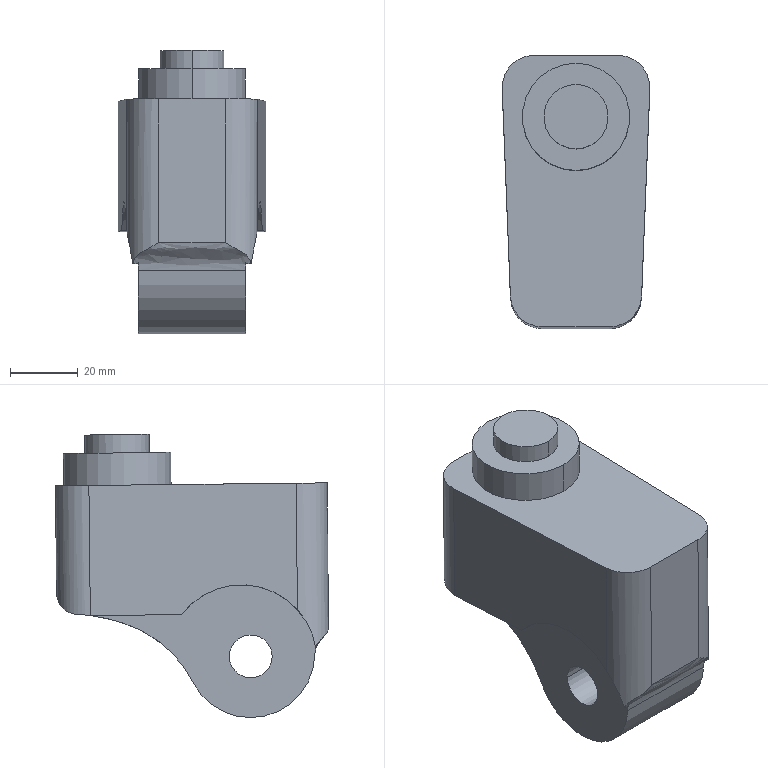Component | NX | CONNECTOR | 1 solid | 27 faces | box 43.68 x 80.82 x 83.81 mm | volume 165748 mm3 | cylinder 14 | plane 11 | spline 2 | commonest cylinder face diameters 19.05 x6 12.7 x3 31.75 x2 44.533 x2 38.1 x1
STEP:
#1=VALUE_REPRESENTATION_ITEM('',COUNT_MEASURE(0.));
#2=(LENGTH_UNIT()NAMED_UNIT(*)SI_UNIT(.MILLI.,.METRE.));
#3=UNCERTAINTY_MEASURE_WITH_UNIT(LENGTH_MEASURE(0.0508),#2,'','');
#4=(NAMED_UNIT(*)PLANE_ANGLE_UNIT()SI_UNIT($,.RADIAN.));
#5=PLANE_ANGLE_MEASURE_WITH_UNIT(PLANE_ANGLE_MEASURE(0.01745),#4);
#6=DIMENSIONAL_EXPONENTS(0.,0.,0.,0.,0.,0.,0.);
#7=(CONVERSION_BASED_UNIT('',#5)NAMED_UNIT(#6)PLANE_ANGLE_UNIT());
#8=(NAMED_UNIT(*)SI_UNIT($,.STERADIAN.)SOLID_ANGLE_UNIT());
#9=(GEOMETRIC_REPRESENTATION_CONTEXT(3)GLOBAL_UNCERTAINTY_ASSIGNED_CONTEXT((#3))GLOBAL_UNIT_ASSIGNED_CONTEXT((#2,#7,#8))REPRESENTATION_CONTEXT('',''));
#10=REPRESENTATION('',(#1),#9);
#11=VALUE_REPRESENTATION_ITEM('',COUNT_MEASURE(0.));
#12=REPRESENTATION('',(#11),#9);
#13=CARTESIAN_POINT('',(0.,0.,0.));
#14=DIRECTION('',(0.,0.,1.));
#15=DIRECTION('',(1.,0.,0.));
#16=AXIS2_PLACEMENT_3D('',#13,#14,#15);
#17=SHAPE_REPRESENTATION('',(#16),#9);
#18=CARTESIAN_POINT('',(-0.,49.153,252.991));
#19=VERTEX_POINT('',#18);
#20=CARTESIAN_POINT('',(-0.,49.095,247.591));
#21=VERTEX_POINT('',#20);
#22=CARTESIAN_POINT('',(-0.,49.371,272.99));
#23=DIRECTION('',(0.,-0.01088,-0.9999));
#24=VECTOR('',#23,1.);
#25=LINE('',#22,#24);
#26=EDGE_CURVE('',#19,#21,#25,.T.);
#27=ORIENTED_EDGE('',*,*,#26,.F.);
#28=CARTESIAN_POINT('',(-0.,30.104,253.198));
#29=VERTEX_POINT('',#28);
#30=CARTESIAN_POINT('',(-0.,39.629,253.095));
#31=DIRECTION('',(0.,-0.01088,-0.9999));
#32=DIRECTION('',(0.,-0.9999,0.01088));
#33=AXIS2_PLACEMENT_3D('',#30,#31,#32);
#34=CIRCLE('',#33,9.525);
#35=EDGE_CURVE('',#19,#29,#34,.T.);
#36=ORIENTED_EDGE('',*,*,#35,.T.);
#37=CARTESIAN_POINT('',(-0.,30.046,247.799));
#38=VERTEX_POINT('',#37);
#39=CARTESIAN_POINT('',(-0.,30.322,273.197));
#40=DIRECTION('',(0.,-0.01088,-0.9999));
#41=VECTOR('',#40,1.);
#42=LINE('',#39,#41);
#43=EDGE_CURVE('',#29,#38,#42,.T.);
#44=ORIENTED_EDGE('',*,*,#43,.T.);
#45=CARTESIAN_POINT('',(-0.,39.57,247.695));
#46=DIRECTION('',(-0.,0.01088,0.9999));
#47=DIRECTION('',(0.,-0.9999,0.01088));
#48=AXIS2_PLACEMENT_3D('',#45,#46,#47);
#49=CIRCLE('',#48,9.525);
#50=EDGE_CURVE('',#38,#21,#49,.T.);
#51=ORIENTED_EDGE('',*,*,#50,.T.);
#52=EDGE_LOOP('',(#27,#36,#44,#51));
#53=FACE_OUTER_BOUND('',#52,.T.);
#54=CARTESIAN_POINT('',(-0.,39.847,273.093));
#55=DIRECTION('',(0.,-0.01088,-0.9999));
#56=DIRECTION('',(0.,-0.9999,0.01088));
#57=AXIS2_PLACEMENT_3D('',#54,#55,#56);
#58=CYLINDRICAL_SURFACE('',#57,9.525);
#59=ADVANCED_FACE('',(#53),#58,.T.);
#60=ORIENTED_EDGE('',*,*,#43,.F.);
#61=CARTESIAN_POINT('',(-0.,39.629,253.095));
#62=DIRECTION('',(0.,-0.01088,-0.9999));
#63=DIRECTION('',(0.,-0.9999,0.01088));
#64=AXIS2_PLACEMENT_3D('',#61,#62,#63);
#65=CIRCLE('',#64,9.525);
#66=EDGE_CURVE('',#29,#19,#65,.T.);
#67=ORIENTED_EDGE('',*,*,#66,.T.);
#68=ORIENTED_EDGE('',*,*,#26,.T.);
#69=CARTESIAN_POINT('',(-0.,39.57,247.695));
#70=DIRECTION('',(-0.,0.01088,0.9999));
#71=DIRECTION('',(0.,-0.9999,0.01088));
#72=AXIS2_PLACEMENT_3D('',#69,#70,#71);
#73=CIRCLE('',#72,9.525);
#74=EDGE_CURVE('',#21,#38,#73,.T.);
#75=ORIENTED_EDGE('',*,*,#74,.T.);
#76=EDGE_LOOP('',(#60,#67,#68,#75));
#77=FACE_OUTER_BOUND('',#76,.T.);
#78=CARTESIAN_POINT('',(-0.,39.847,273.093));
#79=DIRECTION('',(0.,-0.01088,-0.9999));
#80=DIRECTION('',(0.,-0.9999,0.01088));
#81=AXIS2_PLACEMENT_3D('',#78,#79,#80);
#82=CYLINDRICAL_SURFACE('',#81,9.525);
#83=ADVANCED_FACE('',(#77),#82,.T.);
#84=CARTESIAN_POINT('',(-15.875,6.35,187.431));
#85=VERTEX_POINT('',#84);
#86=CARTESIAN_POINT('',(-15.875,-6.35,187.569));
#87=VERTEX_POINT('',#86);
#88=CARTESIAN_POINT('',(-15.875,0.,187.5));
#89=DIRECTION('',(-1.,-0.,-0.));
#90=DIRECTION('',(0.,0.9999,-0.01088));
#91=AXIS2_PLACEMENT_3D('',#88,#89,#90);
#92=CIRCLE('',#91,6.35);
#93=EDGE_CURVE('',#85,#87,#92,.T.);
#94=ORIENTED_EDGE('',*,*,#93,.T.);
#95=CARTESIAN_POINT('',(15.875,-6.35,187.569));
#96=VERTEX_POINT('',#95);
#97=CARTESIAN_POINT('',(-59.055,-6.35,187.569));
#98=DIRECTION('',(1.,0.,0.));
#99=VECTOR('',#98,1.);
#100=LINE('',#97,#99);
#101=EDGE_CURVE('',#87,#96,#100,.T.);
#102=ORIENTED_EDGE('',*,*,#101,.T.);
#103=CARTESIAN_POINT('',(15.875,6.35,187.431));
#104=VERTEX_POINT('',#103);
#105=CARTESIAN_POINT('',(15.875,0.,187.5));
#106=DIRECTION('',(1.,0.,0.));
#107=DIRECTION('',(0.,-0.9999,0.01088));
#108=AXIS2_PLACEMENT_3D('',#105,#106,#107);
#109=CIRCLE('',#108,6.35);
#110=EDGE_CURVE('',#96,#104,#109,.T.);
#111=ORIENTED_EDGE('',*,*,#110,.T.);
#112=CARTESIAN_POINT('',(-59.055,6.35,187.431));
#113=DIRECTION('',(1.,0.,0.));
#114=VECTOR('',#113,1.);
#115=LINE('',#112,#114);
#116=EDGE_CURVE('',#85,#104,#115,.T.);
#117=ORIENTED_EDGE('',*,*,#116,.F.);
#118=EDGE_LOOP('',(#94,#102,#111,#117));
#119=FACE_OUTER_BOUND('',#118,.T.);
#120=CARTESIAN_POINT('',(-59.055,0.,187.5));
#121=DIRECTION('',(1.,0.,0.));
#122=DIRECTION('',(0.,-0.9999,0.01088));
#123=AXIS2_PLACEMENT_3D('',#120,#121,#122);
#124=CYLINDRICAL_SURFACE('',#123,6.35);
#125=ADVANCED_FACE('',(#119),#124,.F.);
#126=CARTESIAN_POINT('',(-0.,23.696,247.868));
#127=VERTEX_POINT('',#126);
#128=CARTESIAN_POINT('',(-0.,55.444,247.522));
#129=VERTEX_POINT('',#128);
#130=CARTESIAN_POINT('',(-0.,39.57,247.695));
#131=DIRECTION('',(-0.,0.01088,0.9999));
#132=DIRECTION('',(0.,-0.9999,0.01088));
#133=AXIS2_PLACEMENT_3D('',#130,#131,#132);
#134=CIRCLE('',#133,15.875);
#135=EDGE_CURVE('',#127,#129,#134,.T.);
#136=ORIENTED_EDGE('',*,*,#135,.F.);
#137=CARTESIAN_POINT('',(-0.,23.592,238.343));
#138=VERTEX_POINT('',#137);
#139=CARTESIAN_POINT('',(-0.,23.696,247.868));
#140=DIRECTION('',(0.,-0.01088,-0.9999));
#141=VECTOR('',#140,1.);
#142=LINE('',#139,#141);
#143=EDGE_CURVE('',#127,#138,#142,.T.);
#144=ORIENTED_EDGE('',*,*,#143,.T.);
#145=CARTESIAN_POINT('',(-0.,55.34,237.998));
#146=VERTEX_POINT('',#145);
#147=CARTESIAN_POINT('',(-0.,39.466,238.17));
#148=DIRECTION('',(-0.,0.01088,0.9999));
#149=DIRECTION('',(0.,0.9999,-0.01088));
#150=AXIS2_PLACEMENT_3D('',#147,#148,#149);
#151=CIRCLE('',#150,15.875);
#152=EDGE_CURVE('',#138,#146,#151,.T.);
#153=ORIENTED_EDGE('',*,*,#152,.T.);
#154=CARTESIAN_POINT('',(-0.,55.444,247.522));
#155=DIRECTION('',(0.,-0.01088,-0.9999));
#156=VECTOR('',#155,1.);
#157=LINE('',#154,#156);
#158=EDGE_CURVE('',#129,#146,#157,.T.);
#159=ORIENTED_EDGE('',*,*,#158,.F.);
#160=EDGE_LOOP('',(#136,#144,#153,#159));
#161=FACE_OUTER_BOUND('',#160,.T.);
#162=CARTESIAN_POINT('',(-0.,39.57,247.695));
#163=DIRECTION('',(0.,-0.01088,-0.9999));
#164=DIRECTION('',(0.,-0.9999,0.01088));
#165=AXIS2_PLACEMENT_3D('',#162,#163,#164);
#166=CYLINDRICAL_SURFACE('',#165,15.875);
#167=ADVANCED_FACE('',(#161),#166,.T.);
#168=CARTESIAN_POINT('',(-15.875,-18.954,188.007));
#169=VERTEX_POINT('',#168);
#170=CARTESIAN_POINT('',(-15.875,17.049,179.757));
#171=VERTEX_POINT('',#170);
#172=CARTESIAN_POINT('',(-15.875,0.09125,188.436));
#173=DIRECTION('',(1.,0.,0.));
#174=DIRECTION('',(0.,0.9999,-0.01088));
#175=AXIS2_PLACEMENT_3D('',#172,#173,#174);
#176=CIRCLE('',#175,19.05);
#177=EDGE_CURVE('',#169,#171,#176,.T.);
#178=ORIENTED_EDGE('',*,*,#177,.F.);
#179=CARTESIAN_POINT('',(-15.875,-19.245,190.037));
#180=VERTEX_POINT('',#179);
#181=CARTESIAN_POINT('',(-15.875,-19.245,190.037));
#182=CARTESIAN_POINT('',(-15.875,-19.078,189.463));
#183=CARTESIAN_POINT('',(-15.875,-18.972,188.797));
#184=CARTESIAN_POINT('',(-15.875,-18.954,188.007));
#185=B_SPLINE_CURVE_WITH_KNOTS('',3,(#181,#182,#183,#184),.UNSPECIFIED.,.F.,.F.,(4,4),(0.,1.),.UNSPECIFIED.);
#186=EDGE_CURVE('',#180,#169,#185,.T.);
#187=ORIENTED_EDGE('',*,*,#186,.F.);
#188=CARTESIAN_POINT('',(-15.875,20.464,199.871));
#189=VERTEX_POINT('',#188);
#190=CARTESIAN_POINT('',(-15.875,2.725,186.414));
#191=DIRECTION('',(1.,0.,0.));
#192=DIRECTION('',(0.,0.9999,-0.01088));
#193=AXIS2_PLACEMENT_3D('',#190,#191,#192);
#194=CIRCLE('',#193,22.266);
#195=EDGE_CURVE('',#189,#180,#194,.T.);
#196=ORIENTED_EDGE('',*,*,#195,.F.);
#197=CARTESIAN_POINT('',(-15.875,47.475,199.577));
#198=VERTEX_POINT('',#197);
#199=CARTESIAN_POINT('',(-15.875,47.475,199.577));
#200=DIRECTION('',(0.,-0.9999,0.01088));
#201=VECTOR('',#200,1.);
#202=LINE('',#199,#201);
#203=EDGE_CURVE('',#198,#189,#202,.T.);
#204=ORIENTED_EDGE('',*,*,#203,.F.);
#205=CARTESIAN_POINT('',(-15.875,17.049,179.757));
#206=CARTESIAN_POINT('',(-15.875,25.735,196.727));
#207=CARTESIAN_POINT('',(-15.875,47.475,199.577));
#208=B_SPLINE_CURVE_WITH_KNOTS('',2,(#205,#206,#207),.UNSPECIFIED.,.F.,.F.,(3,3),(0.,1.),.UNSPECIFIED.);
#209=EDGE_CURVE('',#171,#198,#208,.T.);
#210=ORIENTED_EDGE('',*,*,#209,.F.);
#211=EDGE_LOOP('',(#178,#187,#196,#204,#210));
#212=FACE_BOUND('',#211,.T.);
#213=ORIENTED_EDGE('',*,*,#93,.F.);
#214=CARTESIAN_POINT('',(-15.875,0.,187.5));
#215=DIRECTION('',(-1.,-0.,-0.));
#216=DIRECTION('',(0.,0.9999,-0.01088));
#217=AXIS2_PLACEMENT_3D('',#214,#215,#216);
#218=CIRCLE('',#217,6.35);
#219=EDGE_CURVE('',#87,#85,#218,.T.);
#220=ORIENTED_EDGE('',*,*,#219,.F.);
#221=EDGE_LOOP('',(#213,#220));
#222=FACE_BOUND('',#221,.T.);
#223=CARTESIAN_POINT('',(-15.875,2.725,186.414));
#224=DIRECTION('',(1.,0.,0.));
#225=DIRECTION('',(0.,-0.9999,0.01088));
#226=AXIS2_PLACEMENT_3D('',#223,#224,#225);
#227=PLANE('',#226);
#228=ADVANCED_FACE('',(#212,#222),#227,.F.);
#229=CARTESIAN_POINT('',(15.875,47.475,199.577));
#230=VERTEX_POINT('',#229);
#231=CARTESIAN_POINT('',(15.875,20.464,199.871));
#232=VERTEX_POINT('',#231);
#233=CARTESIAN_POINT('',(15.875,47.475,199.577));
#234=DIRECTION('',(0.,-0.9999,0.01088));
#235=VECTOR('',#234,1.);
#236=LINE('',#233,#235);
#237=EDGE_CURVE('',#230,#232,#236,.T.);
#238=ORIENTED_EDGE('',*,*,#237,.T.);
#239=CARTESIAN_POINT('',(15.875,-19.245,190.037));
#240=VERTEX_POINT('',#239);
#241=CARTESIAN_POINT('',(15.875,2.725,186.414));
#242=DIRECTION('',(1.,0.,0.));
#243=DIRECTION('',(0.,0.9999,-0.01088));
#244=AXIS2_PLACEMENT_3D('',#241,#242,#243);
#245=CIRCLE('',#244,22.266);
#246=EDGE_CURVE('',#232,#240,#245,.T.);
#247=ORIENTED_EDGE('',*,*,#246,.T.);
#248=CARTESIAN_POINT('',(15.875,-18.954,188.007));
#249=VERTEX_POINT('',#248);
#250=CARTESIAN_POINT('',(15.875,-18.954,188.007));
#251=CARTESIAN_POINT('',(15.875,-18.972,188.797));
#252=CARTESIAN_POINT('',(15.875,-19.078,189.463));
#253=CARTESIAN_POINT('',(15.875,-19.245,190.037));
#254=B_SPLINE_CURVE_WITH_KNOTS('',3,(#250,#251,#252,#253),.UNSPECIFIED.,.F.,.F.,(4,4),(0.,1.),.UNSPECIFIED.);
#255=EDGE_CURVE('',#249,#240,#254,.T.);
#256=ORIENTED_EDGE('',*,*,#255,.F.);
#257=CARTESIAN_POINT('',(15.875,17.049,179.757));
#258=VERTEX_POINT('',#257);
#259=CARTESIAN_POINT('',(15.875,0.09125,188.436));
#260=DIRECTION('',(-1.,-0.,-0.));
#261=DIRECTION('',(0.,-0.9999,0.01088));
#262=AXIS2_PLACEMENT_3D('',#259,#260,#261);
#263=CIRCLE('',#262,19.05);
#264=EDGE_CURVE('',#258,#249,#263,.T.);
#265=ORIENTED_EDGE('',*,*,#264,.F.);
#266=CARTESIAN_POINT('',(15.875,47.475,199.577));
#267=CARTESIAN_POINT('',(15.875,25.735,196.727));
#268=CARTESIAN_POINT('',(15.875,17.049,179.757));
#269=B_SPLINE_CURVE_WITH_KNOTS('',2,(#266,#267,#268),.UNSPECIFIED.,.F.,.F.,(3,3),(0.,1.),.UNSPECIFIED.);
#270=EDGE_CURVE('',#230,#258,#269,.T.);
#271=ORIENTED_EDGE('',*,*,#270,.F.);
#272=EDGE_LOOP('',(#238,#247,#256,#265,#271));
#273=FACE_BOUND('',#272,.T.);
#274=CARTESIAN_POINT('',(15.875,0.,187.5));
#275=DIRECTION('',(1.,0.,0.));
#276=DIRECTION('',(0.,-0.9999,0.01088));
#277=AXIS2_PLACEMENT_3D('',#274,#275,#276);
#278=CIRCLE('',#277,6.35);
#279=EDGE_CURVE('',#104,#96,#278,.T.);
#280=ORIENTED_EDGE('',*,*,#279,.F.);
#281=ORIENTED_EDGE('',*,*,#110,.F.);
#282=EDGE_LOOP('',(#280,#281));
#283=FACE_BOUND('',#282,.T.);
#284=CARTESIAN_POINT('',(15.875,2.725,186.414));
#285=DIRECTION('',(-1.,-0.,-0.));
#286=DIRECTION('',(0.,-0.9999,0.01088));
#287=AXIS2_PLACEMENT_3D('',#284,#285,#286);
#288=PLANE('',#287);
#289=ADVANCED_FACE('',(#273,#283),#288,.F.);
#290=CARTESIAN_POINT('',(-0.,39.57,247.695));
#291=DIRECTION('',(-0.,0.01088,0.9999));
#292=DIRECTION('',(0.,-0.9999,0.01088));
#293=AXIS2_PLACEMENT_3D('',#290,#291,#292);
#294=CIRCLE('',#293,15.875);
#295=EDGE_CURVE('',#129,#127,#294,.T.);
#296=ORIENTED_EDGE('',*,*,#295,.T.);
#297=ORIENTED_EDGE('',*,*,#135,.T.);
#298=EDGE_LOOP('',(#296,#297));
#299=FACE_BOUND('',#298,.T.);
#300=ORIENTED_EDGE('',*,*,#74,.F.);
#301=ORIENTED_EDGE('',*,*,#50,.F.);
#302=EDGE_LOOP('',(#300,#301));
#303=FACE_BOUND('',#302,.T.);
#304=CARTESIAN_POINT('',(-0.,39.57,247.695));
#305=DIRECTION('',(-0.,0.01088,0.9999));
#306=DIRECTION('',(0.,0.9999,-0.01088));
#307=AXIS2_PLACEMENT_3D('',#304,#305,#306);
#308=PLANE('',#307);
#309=ADVANCED_FACE('',(#299,#303),#308,.T.);
#310=CARTESIAN_POINT('',(12.316,57.794,237.971));
#311=VERTEX_POINT('',#310);
#312=CARTESIAN_POINT('',(-12.316,57.794,237.971));
#313=VERTEX_POINT('',#312);
#314=CARTESIAN_POINT('',(22.225,57.794,237.971));
#315=DIRECTION('',(-1.,-0.,-0.));
#316=VECTOR('',#315,1.);
#317=LINE('',#314,#316);
#318=EDGE_CURVE('',#311,#313,#317,.T.);
#319=ORIENTED_EDGE('',*,*,#318,.T.);
#320=CARTESIAN_POINT('',(-21.834,47.894,238.079));
#321=VERTEX_POINT('',#320);
#322=CARTESIAN_POINT('',(-12.316,48.27,238.075));
#323=DIRECTION('',(0.,-0.01088,-0.9999));
#324=DIRECTION('',(0.,-0.9999,0.01088));
#325=AXIS2_PLACEMENT_3D('',#322,#323,#324);
#326=CIRCLE('',#325,9.525);
#327=EDGE_CURVE('',#321,#313,#326,.T.);
#328=ORIENTED_EDGE('',*,*,#327,.F.);
#329=CARTESIAN_POINT('',(-19.411,-13.409,238.746));
#330=VERTEX_POINT('',#329);
#331=CARTESIAN_POINT('',(-21.834,47.894,238.079));
#332=DIRECTION('',(-0.03948,0.9992,-0.01088));
#333=VECTOR('',#332,1.);
#334=LINE('',#331,#333);
#335=EDGE_CURVE('',#330,#321,#334,.T.);
#336=ORIENTED_EDGE('',*,*,#335,.F.);
#337=CARTESIAN_POINT('',(-9.894,-22.558,238.846));
#338=VERTEX_POINT('',#337);
#339=CARTESIAN_POINT('',(-9.894,-13.033,238.742));
#340=DIRECTION('',(0.,-0.01088,-0.9999));
#341=DIRECTION('',(0.,0.9999,-0.01088));
#342=AXIS2_PLACEMENT_3D('',#339,#340,#341);
#343=CIRCLE('',#342,9.525);
#344=EDGE_CURVE('',#338,#330,#343,.T.);
#345=ORIENTED_EDGE('',*,*,#344,.F.);
#346=CARTESIAN_POINT('',(9.894,-22.558,238.846));
#347=VERTEX_POINT('',#346);
#348=CARTESIAN_POINT('',(22.225,-22.558,238.846));
#349=DIRECTION('',(-1.,-0.,-0.));
#350=VECTOR('',#349,1.);
#351=LINE('',#348,#350);
#352=EDGE_CURVE('',#347,#338,#351,.T.);
#353=ORIENTED_EDGE('',*,*,#352,.F.);
#354=CARTESIAN_POINT('',(19.411,-13.409,238.746));
#355=VERTEX_POINT('',#354);
#356=CARTESIAN_POINT('',(9.894,-13.033,238.742));
#357=DIRECTION('',(0.,-0.01088,-0.9999));
#358=DIRECTION('',(0.,-0.9999,0.01088));
#359=AXIS2_PLACEMENT_3D('',#356,#357,#358);
#360=CIRCLE('',#359,9.525);
#361=EDGE_CURVE('',#355,#347,#360,.T.);
#362=ORIENTED_EDGE('',*,*,#361,.F.);
#363=CARTESIAN_POINT('',(21.834,47.894,238.079));
#364=VERTEX_POINT('',#363);
#365=CARTESIAN_POINT('',(21.834,47.894,238.079));
#366=DIRECTION('',(-0.03948,-0.9992,0.01088));
#367=VECTOR('',#366,1.);
#368=LINE('',#365,#367);
#369=EDGE_CURVE('',#364,#355,#368,.T.);
#370=ORIENTED_EDGE('',*,*,#369,.F.);
#371=CARTESIAN_POINT('',(12.316,48.27,238.075));
#372=DIRECTION('',(0.,-0.01088,-0.9999));
#373=DIRECTION('',(0.,-0.9999,0.01088));
#374=AXIS2_PLACEMENT_3D('',#371,#372,#373);
#375=CIRCLE('',#374,9.525);
#376=EDGE_CURVE('',#311,#364,#375,.T.);
#377=ORIENTED_EDGE('',*,*,#376,.F.);
#378=EDGE_LOOP('',(#319,#328,#336,#345,#353,#362,#370,#377));
#379=FACE_BOUND('',#378,.T.);
#380=CARTESIAN_POINT('',(-0.,39.466,238.17));
#381=DIRECTION('',(-0.,0.01088,0.9999));
#382=DIRECTION('',(0.,0.9999,-0.01088));
#383=AXIS2_PLACEMENT_3D('',#380,#381,#382);
#384=CIRCLE('',#383,15.875);
#385=EDGE_CURVE('',#146,#138,#384,.T.);
#386=ORIENTED_EDGE('',*,*,#385,.F.);
#387=ORIENTED_EDGE('',*,*,#152,.F.);
#388=EDGE_LOOP('',(#386,#387));
#389=FACE_BOUND('',#388,.T.);
#390=CARTESIAN_POINT('',(22.225,-22.558,238.846));
#391=DIRECTION('',(0.,-0.01088,-0.9999));
#392=DIRECTION('',(0.,-0.9999,0.01088));
#393=AXIS2_PLACEMENT_3D('',#390,#391,#392);
#394=PLANE('',#393);
#395=ADVANCED_FACE('',(#379,#389),#394,.F.);
#396=CARTESIAN_POINT('',(21.296,51.03,199.942));
#397=VERTEX_POINT('',#396);
#398=CARTESIAN_POINT('',(21.834,47.475,199.577));
#399=VERTEX_POINT('',#398);
#400=CARTESIAN_POINT('',(21.296,51.03,199.942));
#401=CARTESIAN_POINT('',(21.704,49.876,199.855));
#402=CARTESIAN_POINT('',(21.882,48.69,199.736));
#403=CARTESIAN_POINT('',(21.834,47.475,199.577));
#404=B_SPLINE_CURVE_WITH_KNOTS('',3,(#400,#401,#402,#403),.UNSPECIFIED.,.F.,.F.,(4,4),(0.,1.),.UNSPECIFIED.);
#405=EDGE_CURVE('',#397,#399,#404,.T.);
#406=ORIENTED_EDGE('',*,*,#405,.T.);
#407=CARTESIAN_POINT('',(15.875,47.475,199.577));
#408=DIRECTION('',(1.,0.,0.));
#409=VECTOR('',#408,1.);
#410=LINE('',#407,#409);
#411=EDGE_CURVE('',#230,#399,#410,.T.);
#412=ORIENTED_EDGE('',*,*,#411,.F.);
#413=ORIENTED_EDGE('',*,*,#270,.T.);
#414=CARTESIAN_POINT('',(22.225,17.049,179.757));
#415=DIRECTION('',(-1.,-0.,-0.));
#416=VECTOR('',#415,1.);
#417=LINE('',#414,#416);
#418=EDGE_CURVE('',#258,#171,#417,.T.);
#419=ORIENTED_EDGE('',*,*,#418,.T.);
#420=ORIENTED_EDGE('',*,*,#209,.T.);
#421=CARTESIAN_POINT('',(-21.834,47.475,199.577));
#422=VERTEX_POINT('',#421);
#423=CARTESIAN_POINT('',(-15.875,47.475,199.577));
#424=DIRECTION('',(-1.,-0.,-0.));
#425=VECTOR('',#424,1.);
#426=LINE('',#423,#425);
#427=EDGE_CURVE('',#198,#422,#426,.T.);
#428=ORIENTED_EDGE('',*,*,#427,.T.);
#429=CARTESIAN_POINT('',(-21.296,51.03,199.942));
#430=VERTEX_POINT('',#429);
#431=CARTESIAN_POINT('',(-21.834,47.475,199.577));
#432=CARTESIAN_POINT('',(-21.882,48.69,199.736));
#433=CARTESIAN_POINT('',(-21.704,49.876,199.855));
#434=CARTESIAN_POINT('',(-21.296,51.03,199.942));
#435=B_SPLINE_CURVE_WITH_KNOTS('',3,(#431,#432,#433,#434),.UNSPECIFIED.,.F.,.F.,(4,4),(0.,1.),.UNSPECIFIED.);
#436=EDGE_CURVE('',#422,#430,#435,.T.);
#437=ORIENTED_EDGE('',*,*,#436,.T.);
#438=CARTESIAN_POINT('',(22.225,51.03,199.942));
#439=DIRECTION('',(-1.,-0.,-0.));
#440=VECTOR('',#439,1.);
#441=LINE('',#438,#440);
#442=EDGE_CURVE('',#397,#430,#441,.T.);
#443=ORIENTED_EDGE('',*,*,#442,.F.);
#444=EDGE_LOOP('',(#406,#412,#413,#419,#420,#428,#437,#443));
#445=FACE_OUTER_BOUND('',#444,.T.);
#446=CARTESIAN_POINT('',(22.12,17.049,179.757));
#447=CARTESIAN_POINT('',(-22.12,17.049,179.757));
#448=CARTESIAN_POINT('',(22.12,26.428,198.082));
#449=CARTESIAN_POINT('',(-22.12,26.428,198.082));
#450=CARTESIAN_POINT('',(22.12,51.03,199.942));
#451=CARTESIAN_POINT('',(-22.12,51.03,199.942));
#452=B_SPLINE_SURFACE_WITH_KNOTS('',2,1,((#446,#447),(#448,#449),(#450,#451)),.UNSPECIFIED.,.F.,.F.,.F.,(3,3),(2,2),(0.,1.),(0.,1.),.UNSPECIFIED.);
#453=ADVANCED_FACE('',(#445),#452,.F.);
#454=ORIENTED_EDGE('',*,*,#255,.T.);
#455=CARTESIAN_POINT('',(17.539,-19.245,190.037));
#456=VERTEX_POINT('',#455);
#457=CARTESIAN_POINT('',(15.875,-19.245,190.037));
#458=DIRECTION('',(1.,0.,0.));
#459=VECTOR('',#458,1.);
#460=LINE('',#457,#459);
#461=EDGE_CURVE('',#240,#456,#460,.T.);
#462=ORIENTED_EDGE('',*,*,#461,.T.);
#463=CARTESIAN_POINT('',(9.894,-23.021,196.315));
#464=VERTEX_POINT('',#463);
#465=CARTESIAN_POINT('',(17.539,-19.245,190.037));
#466=CARTESIAN_POINT('',(17.324,-19.524,190.997));
#467=CARTESIAN_POINT('',(16.947,-19.983,191.701));
#468=CARTESIAN_POINT('',(16.213,-20.671,192.523));
#469=CARTESIAN_POINT('',(15.933,-20.91,192.77));
#470=CARTESIAN_POINT('',(15.458,-21.263,193.122));
#471=CARTESIAN_POINT('',(15.291,-21.38,193.237));
#472=CARTESIAN_POINT('',(14.939,-21.609,193.463));
#473=CARTESIAN_POINT('',(14.721,-21.739,193.594));
#474=CARTESIAN_POINT('',(14.236,-22.008,193.874));
#475=CARTESIAN_POINT('',(13.884,-22.179,194.064));
#476=CARTESIAN_POINT('',(13.311,-22.41,194.369));
#477=CARTESIAN_POINT('',(13.113,-22.483,194.474));
#478=CARTESIAN_POINT('',(12.701,-22.618,194.692));
#479=CARTESIAN_POINT('',(12.441,-22.691,194.831));
#480=CARTESIAN_POINT('',(11.575,-22.909,195.299));
#481=CARTESIAN_POINT('',(10.784,-23.027,195.74));
#482=CARTESIAN_POINT('',(9.894,-23.021,196.315));
#483=B_SPLINE_CURVE_WITH_KNOTS('',3,(#465,#466,#467,#468,#469,#470,#471,#472,#473,#474,#475,#476,#477,#478,#479,#480,#481,#482),.UNSPECIFIED.,.F.,.F.,(4,2,2,2,2,2,2,2,4),(0.,0.25,0.375,0.4375,0.5,0.625,0.6875,0.75,1.),.UNSPECIFIED.);
#484=EDGE_CURVE('',#456,#464,#483,.T.);
#485=ORIENTED_EDGE('',*,*,#484,.T.);
#486=CARTESIAN_POINT('',(-9.894,-23.021,196.315));
#487=VERTEX_POINT('',#486);
#488=CARTESIAN_POINT('',(22.225,-23.021,196.315));
#489=DIRECTION('',(-1.,-0.,-0.));
#490=VECTOR('',#489,1.);
#491=LINE('',#488,#490);
#492=EDGE_CURVE('',#464,#487,#491,.T.);
#493=ORIENTED_EDGE('',*,*,#492,.T.);
#494=CARTESIAN_POINT('',(-17.539,-19.245,190.037));
#495=VERTEX_POINT('',#494);
#496=CARTESIAN_POINT('',(-9.894,-23.021,196.315));
#497=CARTESIAN_POINT('',(-10.339,-23.024,196.028));
#498=CARTESIAN_POINT('',(-10.759,-22.995,195.774));
#499=CARTESIAN_POINT('',(-11.353,-22.92,195.431));
#500=CARTESIAN_POINT('',(-11.544,-22.889,195.322));
#501=CARTESIAN_POINT('',(-11.915,-22.818,195.116));
#502=CARTESIAN_POINT('',(-12.048,-22.79,195.043));
#503=CARTESIAN_POINT('',(-12.709,-22.624,194.686));
#504=CARTESIAN_POINT('',(-13.12,-22.487,194.471));
#505=CARTESIAN_POINT('',(-13.693,-22.256,194.166));
#506=CARTESIAN_POINT('',(-13.876,-22.175,194.068));
#507=CARTESIAN_POINT('',(-14.229,-22.006,193.875));
#508=CARTESIAN_POINT('',(-14.365,-21.936,193.799));
#509=CARTESIAN_POINT('',(-16.113,-20.965,192.788));
#510=CARTESIAN_POINT('',(-17.108,-19.804,191.957));
#511=CARTESIAN_POINT('',(-17.539,-19.245,190.037));
#512=B_SPLINE_CURVE_WITH_KNOTS('',3,(#496,#497,#498,#499,#500,#501,#502,#503,#504,#505,#506,#507,#508,#509,#510,#511),.UNSPECIFIED.,.F.,.F.,(4,2,2,2,2,2,2,4),(0.,0.125,0.1875,0.25,0.375,0.4375,0.5,1.),.UNSPECIFIED.);
#513=EDGE_CURVE('',#487,#495,#512,.T.);
#514=ORIENTED_EDGE('',*,*,#513,.T.);
#515=CARTESIAN_POINT('',(-15.875,-19.245,190.037));
#516=DIRECTION('',(-1.,-0.,-0.));
#517=VECTOR('',#516,1.);
#518=LINE('',#515,#517);
#519=EDGE_CURVE('',#180,#495,#518,.T.);
#520=ORIENTED_EDGE('',*,*,#519,.F.);
#521=ORIENTED_EDGE('',*,*,#186,.T.);
#522=CARTESIAN_POINT('',(22.225,-18.954,188.007));
#523=DIRECTION('',(-1.,-0.,-0.));
#524=VECTOR('',#523,1.);
#525=LINE('',#522,#524);
#526=EDGE_CURVE('',#249,#169,#525,.T.);
#527=ORIENTED_EDGE('',*,*,#526,.F.);
#528=EDGE_LOOP('',(#454,#462,#485,#493,#514,#520,#521,#527));
#529=FACE_OUTER_BOUND('',#528,.T.);
#530=CARTESIAN_POINT('',(17.75,-23.021,196.315));
#531=CARTESIAN_POINT('',(-17.75,-23.021,196.315));
#532=CARTESIAN_POINT('',(17.75,-23.056,193.067));
#533=CARTESIAN_POINT('',(-17.75,-23.056,193.067));
#534=CARTESIAN_POINT('',(17.75,-19.072,193.235));
#535=CARTESIAN_POINT('',(-17.75,-19.072,193.235));
#536=CARTESIAN_POINT('',(17.75,-18.954,188.007));
#537=CARTESIAN_POINT('',(-17.75,-18.954,188.007));
#538=B_SPLINE_SURFACE_WITH_KNOTS('',3,1,((#530,#531),(#532,#533),(#534,#535),(#536,#537)),.UNSPECIFIED.,.F.,.F.,.F.,(4,4),(2,2),(0.,1.),(0.,1.),.UNSPECIFIED.);
#539=ADVANCED_FACE('',(#529),#538,.F.);
#540=CARTESIAN_POINT('',(-20.767,20.464,199.871));
#541=VERTEX_POINT('',#540);
#542=CARTESIAN_POINT('',(-21.834,47.475,199.577));
#543=DIRECTION('',(-0.03948,0.9992,-0.01088));
#544=VECTOR('',#543,1.);
#545=LINE('',#542,#544);
#546=EDGE_CURVE('',#541,#422,#545,.T.);
#547=ORIENTED_EDGE('',*,*,#546,.F.);
#548=CARTESIAN_POINT('',(-19.411,-13.817,201.319));
#549=VERTEX_POINT('',#548);
#550=CARTESIAN_POINT('',(-19.411,-13.817,201.319));
#551=CARTESIAN_POINT('',(-19.806,-3.72,212.523));
#552=CARTESIAN_POINT('',(-20.401,11.349,211.887));
#553=CARTESIAN_POINT('',(-20.767,20.464,199.871));
#554=(BOUNDED_CURVE()B_SPLINE_CURVE(3,(#550,#551,#552,#553),.UNSPECIFIED.,.F.,.F.)B_SPLINE_CURVE_WITH_KNOTS((4,4),(0.,1.),.UNSPECIFIED.)CURVE()GEOMETRIC_REPRESENTATION_ITEM()RATIONAL_B_SPLINE_CURVE((1.,0.7583,0.7583,1.))REPRESENTATION_ITEM(''));
#555=EDGE_CURVE('',#549,#541,#554,.T.);
#556=ORIENTED_EDGE('',*,*,#555,.F.);
#557=CARTESIAN_POINT('',(-19.411,-14.316,155.439));
#558=DIRECTION('',(-0.,0.01088,0.9999));
#559=VECTOR('',#558,1.);
#560=LINE('',#557,#559);
#561=EDGE_CURVE('',#549,#330,#560,.T.);
#562=ORIENTED_EDGE('',*,*,#561,.T.);
#563=ORIENTED_EDGE('',*,*,#335,.T.);
#564=CARTESIAN_POINT('',(-21.834,46.987,154.772));
#565=DIRECTION('',(-0.,0.01088,0.9999));
#566=VECTOR('',#565,1.);
#567=LINE('',#564,#566);
#568=EDGE_CURVE('',#422,#321,#567,.T.);
#569=ORIENTED_EDGE('',*,*,#568,.F.);
#570=EDGE_LOOP('',(#547,#556,#562,#563,#569));
#571=FACE_OUTER_BOUND('',#570,.T.);
#572=CARTESIAN_POINT('',(-21.834,46.987,154.772));
#573=DIRECTION('',(0.9992,0.03948,-0.0004297));
#574=DIRECTION('',(0.03948,-0.9992,0.01088));
#575=AXIS2_PLACEMENT_3D('',#572,#573,#574);
#576=PLANE('',#575);
#577=ADVANCED_FACE('',(#571),#576,.F.);
#578=CARTESIAN_POINT('',(-17.539,-19.245,190.037));
#579=CARTESIAN_POINT('',(-18.024,-18.546,194.271));
#580=CARTESIAN_POINT('',(-19.299,-16.709,198.11));
#581=CARTESIAN_POINT('',(-19.411,-13.817,201.319));
#582=B_SPLINE_CURVE_WITH_KNOTS('',3,(#578,#579,#580,#581),.UNSPECIFIED.,.F.,.F.,(4,4),(0.,1.),.UNSPECIFIED.);
#583=EDGE_CURVE('',#495,#549,#582,.T.);
#584=ORIENTED_EDGE('',*,*,#583,.F.);
#585=ORIENTED_EDGE('',*,*,#513,.F.);
#586=CARTESIAN_POINT('',(-9.894,-23.464,155.539));
#587=DIRECTION('',(-0.,0.01088,0.9999));
#588=VECTOR('',#587,1.);
#589=LINE('',#586,#588);
#590=EDGE_CURVE('',#487,#338,#589,.T.);
#591=ORIENTED_EDGE('',*,*,#590,.T.);
#592=ORIENTED_EDGE('',*,*,#344,.T.);
#593=ORIENTED_EDGE('',*,*,#561,.F.);
#594=EDGE_LOOP('',(#584,#585,#591,#592,#593));
#595=FACE_OUTER_BOUND('',#594,.T.);
#596=CARTESIAN_POINT('',(-9.894,-13.94,155.435));
#597=DIRECTION('',(-0.,0.01088,0.9999));
#598=DIRECTION('',(0.,0.9999,-0.01088));
#599=AXIS2_PLACEMENT_3D('',#596,#597,#598);
#600=CYLINDRICAL_SURFACE('',#599,9.525);
#601=ADVANCED_FACE('',(#595),#600,.T.);
#602=CARTESIAN_POINT('',(-12.316,57.449,206.223));
#603=VERTEX_POINT('',#602);
#604=CARTESIAN_POINT('',(-12.316,56.888,154.664));
#605=DIRECTION('',(-0.,0.01088,0.9999));
#606=VECTOR('',#605,1.);
#607=LINE('',#604,#606);
#608=EDGE_CURVE('',#603,#313,#607,.T.);
#609=ORIENTED_EDGE('',*,*,#608,.T.);
#610=ORIENTED_EDGE('',*,*,#318,.F.);
#611=CARTESIAN_POINT('',(12.316,57.449,206.223));
#612=VERTEX_POINT('',#611);
#613=CARTESIAN_POINT('',(12.316,56.888,154.664));
#614=DIRECTION('',(-0.,0.01088,0.9999));
#615=VECTOR('',#614,1.);
#616=LINE('',#613,#615);
#617=EDGE_CURVE('',#612,#311,#616,.T.);
#618=ORIENTED_EDGE('',*,*,#617,.F.);
#619=CARTESIAN_POINT('',(22.225,57.449,206.223));
#620=DIRECTION('',(-1.,-0.,-0.));
#621=VECTOR('',#620,1.);
#622=LINE('',#619,#621);
#623=EDGE_CURVE('',#612,#603,#622,.T.);
#624=ORIENTED_EDGE('',*,*,#623,.T.);
#625=EDGE_LOOP('',(#609,#610,#618,#624));
#626=FACE_OUTER_BOUND('',#625,.T.);
#627=CARTESIAN_POINT('',(22.225,57.449,206.223));
#628=DIRECTION('',(0.,-0.9999,0.01088));
#629=DIRECTION('',(-1.,0.,0.));
#630=AXIS2_PLACEMENT_3D('',#627,#628,#629);
#631=PLANE('',#630);
#632=ADVANCED_FACE('',(#626),#631,.F.);
#633=ORIENTED_EDGE('',*,*,#352,.T.);
#634=ORIENTED_EDGE('',*,*,#590,.F.);
#635=ORIENTED_EDGE('',*,*,#492,.F.);
#636=CARTESIAN_POINT('',(9.894,-23.464,155.539));
#637=DIRECTION('',(-0.,0.01088,0.9999));
#638=VECTOR('',#637,1.);
#639=LINE('',#636,#638);
#640=EDGE_CURVE('',#464,#347,#639,.T.);
#641=ORIENTED_EDGE('',*,*,#640,.T.);
#642=EDGE_LOOP('',(#633,#634,#635,#641));
#643=FACE_OUTER_BOUND('',#642,.T.);
#644=CARTESIAN_POINT('',(22.225,-22.558,238.846));
#645=DIRECTION('',(0.,0.9999,-0.01088));
#646=DIRECTION('',(1.,0.,0.));
#647=AXIS2_PLACEMENT_3D('',#644,#645,#646);
#648=PLANE('',#647);
#649=ADVANCED_FACE('',(#643),#648,.F.);
#650=ORIENTED_EDGE('',*,*,#442,.T.);
#651=CARTESIAN_POINT('',(-21.296,51.03,199.942));
#652=CARTESIAN_POINT('',(-20.53,53.197,199.919));
#653=CARTESIAN_POINT('',(-19.036,54.879,200.949));
#654=CARTESIAN_POINT('',(-15.833,56.946,203.351));
#655=CARTESIAN_POINT('',(-14.066,57.433,204.794));
#656=CARTESIAN_POINT('',(-12.316,57.449,206.223));
#657=B_SPLINE_CURVE_WITH_KNOTS('',3,(#651,#652,#653,#654,#655,#656),.UNSPECIFIED.,.F.,.F.,(4,2,4),(0.,0.5,1.),.UNSPECIFIED.);
#658=EDGE_CURVE('',#430,#603,#657,.T.);
#659=ORIENTED_EDGE('',*,*,#658,.T.);
#660=ORIENTED_EDGE('',*,*,#623,.F.);
#661=CARTESIAN_POINT('',(12.316,57.449,206.223));
#662=CARTESIAN_POINT('',(14.066,57.433,204.794));
#663=CARTESIAN_POINT('',(15.833,56.946,203.351));
#664=CARTESIAN_POINT('',(19.036,54.879,200.949));
#665=CARTESIAN_POINT('',(20.53,53.197,199.919));
#666=CARTESIAN_POINT('',(21.296,51.03,199.942));
#667=B_SPLINE_CURVE_WITH_KNOTS('',3,(#661,#662,#663,#664,#665,#666),.UNSPECIFIED.,.F.,.F.,(4,2,4),(0.,0.5,1.),.UNSPECIFIED.);
#668=EDGE_CURVE('',#612,#397,#667,.T.);
#669=ORIENTED_EDGE('',*,*,#668,.T.);
#670=EDGE_LOOP('',(#650,#659,#660,#669));
#671=FACE_OUTER_BOUND('',#670,.T.);
#672=CARTESIAN_POINT('',(22.225,51.099,206.292));
#673=DIRECTION('',(-1.,-0.,-0.));
#674=DIRECTION('',(0.,0.9999,-0.01088));
#675=AXIS2_PLACEMENT_3D('',#672,#673,#674);
#676=CYLINDRICAL_SURFACE('',#675,6.35);
#677=ADVANCED_FACE('',(#671),#676,.T.);
#678=ORIENTED_EDGE('',*,*,#418,.F.);
#679=ORIENTED_EDGE('',*,*,#264,.T.);
#680=ORIENTED_EDGE('',*,*,#526,.T.);
#681=ORIENTED_EDGE('',*,*,#177,.T.);
#682=EDGE_LOOP('',(#678,#679,#680,#681));
#683=FACE_OUTER_BOUND('',#682,.T.);
#684=CARTESIAN_POINT('',(22.225,0.09125,188.436));
#685=DIRECTION('',(-1.,-0.,-0.));
#686=DIRECTION('',(0.,0.9999,-0.01088));
#687=AXIS2_PLACEMENT_3D('',#684,#685,#686);
#688=CYLINDRICAL_SURFACE('',#687,19.05);
#689=ADVANCED_FACE('',(#683),#688,.T.);
#690=ORIENTED_EDGE('',*,*,#668,.F.);
#691=ORIENTED_EDGE('',*,*,#617,.T.);
#692=ORIENTED_EDGE('',*,*,#376,.T.);
#693=CARTESIAN_POINT('',(21.834,46.987,154.772));
#694=DIRECTION('',(-0.,0.01088,0.9999));
#695=VECTOR('',#694,1.);
#696=LINE('',#693,#695);
#697=EDGE_CURVE('',#399,#364,#696,.T.);
#698=ORIENTED_EDGE('',*,*,#697,.F.);
#699=ORIENTED_EDGE('',*,*,#405,.F.);
#700=EDGE_LOOP('',(#690,#691,#692,#698,#699));
#701=FACE_OUTER_BOUND('',#700,.T.);
#702=CARTESIAN_POINT('',(12.316,47.363,154.768));
#703=DIRECTION('',(-0.,0.01088,0.9999));
#704=DIRECTION('',(0.,0.9999,-0.01088));
#705=AXIS2_PLACEMENT_3D('',#702,#703,#704);
#706=CYLINDRICAL_SURFACE('',#705,9.525);
#707=ADVANCED_FACE('',(#701),#706,.T.);
#708=ORIENTED_EDGE('',*,*,#484,.F.);
#709=CARTESIAN_POINT('',(19.411,-13.817,201.319));
#710=VERTEX_POINT('',#709);
#711=CARTESIAN_POINT('',(17.539,-19.245,190.037));
#712=CARTESIAN_POINT('',(18.024,-18.546,194.271));
#713=CARTESIAN_POINT('',(19.299,-16.709,198.11));
#714=CARTESIAN_POINT('',(19.411,-13.817,201.319));
#715=B_SPLINE_CURVE_WITH_KNOTS('',3,(#711,#712,#713,#714),.UNSPECIFIED.,.F.,.F.,(4,4),(0.,1.),.UNSPECIFIED.);
#716=EDGE_CURVE('',#456,#710,#715,.T.);
#717=ORIENTED_EDGE('',*,*,#716,.T.);
#718=CARTESIAN_POINT('',(19.411,-14.316,155.439));
#719=DIRECTION('',(-0.,0.01088,0.9999));
#720=VECTOR('',#719,1.);
#721=LINE('',#718,#720);
#722=EDGE_CURVE('',#710,#355,#721,.T.);
#723=ORIENTED_EDGE('',*,*,#722,.T.);
#724=ORIENTED_EDGE('',*,*,#361,.T.);
#725=ORIENTED_EDGE('',*,*,#640,.F.);
#726=EDGE_LOOP('',(#708,#717,#723,#724,#725));
#727=FACE_OUTER_BOUND('',#726,.T.);
#728=CARTESIAN_POINT('',(9.894,-13.94,155.435));
#729=DIRECTION('',(-0.,0.01088,0.9999));
#730=DIRECTION('',(0.,0.9999,-0.01088));
#731=AXIS2_PLACEMENT_3D('',#728,#729,#730);
#732=CYLINDRICAL_SURFACE('',#731,9.525);
#733=ADVANCED_FACE('',(#727),#732,.T.);
#734=ORIENTED_EDGE('',*,*,#722,.F.);
#735=CARTESIAN_POINT('',(20.767,20.464,199.871));
#736=VERTEX_POINT('',#735);
#737=CARTESIAN_POINT('',(19.411,-13.817,201.319));
#738=CARTESIAN_POINT('',(19.806,-3.72,212.523));
#739=CARTESIAN_POINT('',(20.401,11.349,211.887));
#740=CARTESIAN_POINT('',(20.767,20.464,199.871));
#741=(BOUNDED_CURVE()B_SPLINE_CURVE(3,(#737,#738,#739,#740),.UNSPECIFIED.,.F.,.F.)B_SPLINE_CURVE_WITH_KNOTS((4,4),(0.,1.),.UNSPECIFIED.)CURVE()GEOMETRIC_REPRESENTATION_ITEM()RATIONAL_B_SPLINE_CURVE((1.,0.7583,0.7583,1.))REPRESENTATION_ITEM(''));
#742=EDGE_CURVE('',#710,#736,#741,.T.);
#743=ORIENTED_EDGE('',*,*,#742,.T.);
#744=CARTESIAN_POINT('',(21.834,47.475,199.577));
#745=DIRECTION('',(0.03948,0.9992,-0.01088));
#746=VECTOR('',#745,1.);
#747=LINE('',#744,#746);
#748=EDGE_CURVE('',#736,#399,#747,.T.);
#749=ORIENTED_EDGE('',*,*,#748,.T.);
#750=ORIENTED_EDGE('',*,*,#697,.T.);
#751=ORIENTED_EDGE('',*,*,#369,.T.);
#752=EDGE_LOOP('',(#734,#743,#749,#750,#751));
#753=FACE_OUTER_BOUND('',#752,.T.);
#754=CARTESIAN_POINT('',(21.834,46.987,154.772));
#755=DIRECTION('',(-0.9992,0.03948,-0.0004297));
#756=DIRECTION('',(0.03948,0.9992,-0.01088));
#757=AXIS2_PLACEMENT_3D('',#754,#755,#756);
#758=PLANE('',#757);
#759=ADVANCED_FACE('',(#753),#758,.F.);
#760=ORIENTED_EDGE('',*,*,#568,.T.);
#761=ORIENTED_EDGE('',*,*,#327,.T.);
#762=ORIENTED_EDGE('',*,*,#608,.F.);
#763=ORIENTED_EDGE('',*,*,#658,.F.);
#764=ORIENTED_EDGE('',*,*,#436,.F.);
#765=EDGE_LOOP('',(#760,#761,#762,#763,#764));
#766=FACE_OUTER_BOUND('',#765,.T.);
#767=CARTESIAN_POINT('',(-12.316,47.363,154.768));
#768=DIRECTION('',(-0.,0.01088,0.9999));
#769=DIRECTION('',(0.,0.9999,-0.01088));
#770=AXIS2_PLACEMENT_3D('',#767,#768,#769);
#771=CYLINDRICAL_SURFACE('',#770,9.525);
#772=ADVANCED_FACE('',(#766),#771,.T.);
#773=ORIENTED_EDGE('',*,*,#546,.T.);
#774=ORIENTED_EDGE('',*,*,#427,.F.);
#775=ORIENTED_EDGE('',*,*,#203,.T.);
#776=CARTESIAN_POINT('',(-15.875,20.464,199.871));
#777=DIRECTION('',(-1.,-0.,-0.));
#778=VECTOR('',#777,1.);
#779=LINE('',#776,#778);
#780=EDGE_CURVE('',#189,#541,#779,.T.);
#781=ORIENTED_EDGE('',*,*,#780,.T.);
#782=EDGE_LOOP('',(#773,#774,#775,#781));
#783=FACE_OUTER_BOUND('',#782,.T.);
#784=CARTESIAN_POINT('',(-15.875,47.475,199.577));
#785=DIRECTION('',(-0.,-0.01088,-0.9999));
#786=DIRECTION('',(0.,-0.9999,0.01088));
#787=AXIS2_PLACEMENT_3D('',#784,#785,#786);
#788=PLANE('',#787);
#789=ADVANCED_FACE('',(#783),#788,.T.);
#790=ORIENTED_EDGE('',*,*,#555,.T.);
#791=ORIENTED_EDGE('',*,*,#780,.F.);
#792=ORIENTED_EDGE('',*,*,#195,.T.);
#793=ORIENTED_EDGE('',*,*,#519,.T.);
#794=ORIENTED_EDGE('',*,*,#583,.T.);
#795=EDGE_LOOP('',(#790,#791,#792,#793,#794));
#796=FACE_OUTER_BOUND('',#795,.T.);
#797=CARTESIAN_POINT('',(-15.875,2.725,186.414));
#798=DIRECTION('',(-1.,-0.,-0.));
#799=DIRECTION('',(0.,0.9999,-0.01088));
#800=AXIS2_PLACEMENT_3D('',#797,#798,#799);
#801=CYLINDRICAL_SURFACE('',#800,22.266);
#802=ADVANCED_FACE('',(#796),#801,.F.);
#803=ORIENTED_EDGE('',*,*,#461,.F.);
#804=ORIENTED_EDGE('',*,*,#246,.F.);
#805=CARTESIAN_POINT('',(15.875,20.464,199.871));
#806=DIRECTION('',(1.,0.,0.));
#807=VECTOR('',#806,1.);
#808=LINE('',#805,#807);
#809=EDGE_CURVE('',#232,#736,#808,.T.);
#810=ORIENTED_EDGE('',*,*,#809,.T.);
#811=ORIENTED_EDGE('',*,*,#742,.F.);
#812=ORIENTED_EDGE('',*,*,#716,.F.);
#813=EDGE_LOOP('',(#803,#804,#810,#811,#812));
#814=FACE_OUTER_BOUND('',#813,.T.);
#815=CARTESIAN_POINT('',(15.875,2.725,186.414));
#816=DIRECTION('',(1.,0.,0.));
#817=DIRECTION('',(0.,-0.9999,0.01088));
#818=AXIS2_PLACEMENT_3D('',#815,#816,#817);
#819=CYLINDRICAL_SURFACE('',#818,22.266);
#820=ADVANCED_FACE('',(#814),#819,.F.);
#821=ORIENTED_EDGE('',*,*,#809,.F.);
#822=ORIENTED_EDGE('',*,*,#237,.F.);
#823=ORIENTED_EDGE('',*,*,#411,.T.);
#824=ORIENTED_EDGE('',*,*,#748,.F.);
#825=EDGE_LOOP('',(#821,#822,#823,#824));
#826=FACE_OUTER_BOUND('',#825,.T.);
#827=CARTESIAN_POINT('',(15.875,47.475,199.577));
#828=DIRECTION('',(0.,0.01088,0.9999));
#829=DIRECTION('',(0.,0.9999,-0.01088));
#830=AXIS2_PLACEMENT_3D('',#827,#828,#829);
#831=PLANE('',#830);
#832=ADVANCED_FACE('',(#826),#831,.F.);
#833=ORIENTED_EDGE('',*,*,#143,.F.);
#834=ORIENTED_EDGE('',*,*,#295,.F.);
#835=ORIENTED_EDGE('',*,*,#158,.T.);
#836=ORIENTED_EDGE('',*,*,#385,.T.);
#837=EDGE_LOOP('',(#833,#834,#835,#836));
#838=FACE_OUTER_BOUND('',#837,.T.);
#839=CARTESIAN_POINT('',(-0.,39.57,247.695));
#840=DIRECTION('',(0.,-0.01088,-0.9999));
#841=DIRECTION('',(0.,-0.9999,0.01088));
#842=AXIS2_PLACEMENT_3D('',#839,#840,#841);
#843=CYLINDRICAL_SURFACE('',#842,15.875);
#844=ADVANCED_FACE('',(#838),#843,.T.);
#845=ORIENTED_EDGE('',*,*,#101,.F.);
#846=ORIENTED_EDGE('',*,*,#219,.T.);
#847=ORIENTED_EDGE('',*,*,#116,.T.);
#848=ORIENTED_EDGE('',*,*,#279,.T.);
#849=EDGE_LOOP('',(#845,#846,#847,#848));
#850=FACE_OUTER_BOUND('',#849,.T.);
#851=CARTESIAN_POINT('',(-59.055,0.,187.5));
#852=DIRECTION('',(1.,0.,0.));
#853=DIRECTION('',(0.,-0.9999,0.01088));
#854=AXIS2_PLACEMENT_3D('',#851,#852,#853);
#855=CYLINDRICAL_SURFACE('',#854,6.35);
#856=ADVANCED_FACE('',(#850),#855,.F.);
#857=ORIENTED_EDGE('',*,*,#66,.F.);
#858=ORIENTED_EDGE('',*,*,#35,.F.);
#859=EDGE_LOOP('',(#857,#858));
#860=FACE_OUTER_BOUND('',#859,.T.);
#861=CARTESIAN_POINT('',(-0.,39.629,253.095));
#862=DIRECTION('',(0.,0.01088,0.9999));
#863=DIRECTION('',(0.,-0.9999,0.01088));
#864=AXIS2_PLACEMENT_3D('',#861,#862,#863);
#865=PLANE('',#864);
#866=ADVANCED_FACE('',(#860),#865,.T.);
#867=CLOSED_SHELL('',(#59,#83,#125,#167,#228,#289,#309,#395,#453,#539,#577,#601,#632,#649,#677,#689,#707,#733,#759,#772,#789,#802,#820,#832,#844,#856,#866));
#868=MANIFOLD_SOLID_BREP('',#867);
#869=ADVANCED_BREP_SHAPE_REPRESENTATION('',(#868),#9);
#870=SHAPE_REPRESENTATION_RELATIONSHIP('','',#17,#869);
#871=PRESENTATION_LAYER_ASSIGNMENT('','',(#868));
#872=COLOUR_RGB('',1.,0.6,0.);
#873=FILL_AREA_STYLE_COLOUR('',#872);
#874=FILL_AREA_STYLE('',(#873));
#875=SURFACE_STYLE_FILL_AREA(#874);
#876=SURFACE_SIDE_STYLE('',(#875));
#877=SURFACE_STYLE_USAGE(.BOTH.,#876);
#878=PRESENTATION_STYLE_ASSIGNMENT((#877));
#879=STYLED_ITEM('',(#878),#868);
#880=MECHANICAL_DESIGN_GEOMETRIC_PRESENTATION_REPRESENTATION('',(#879),#9);